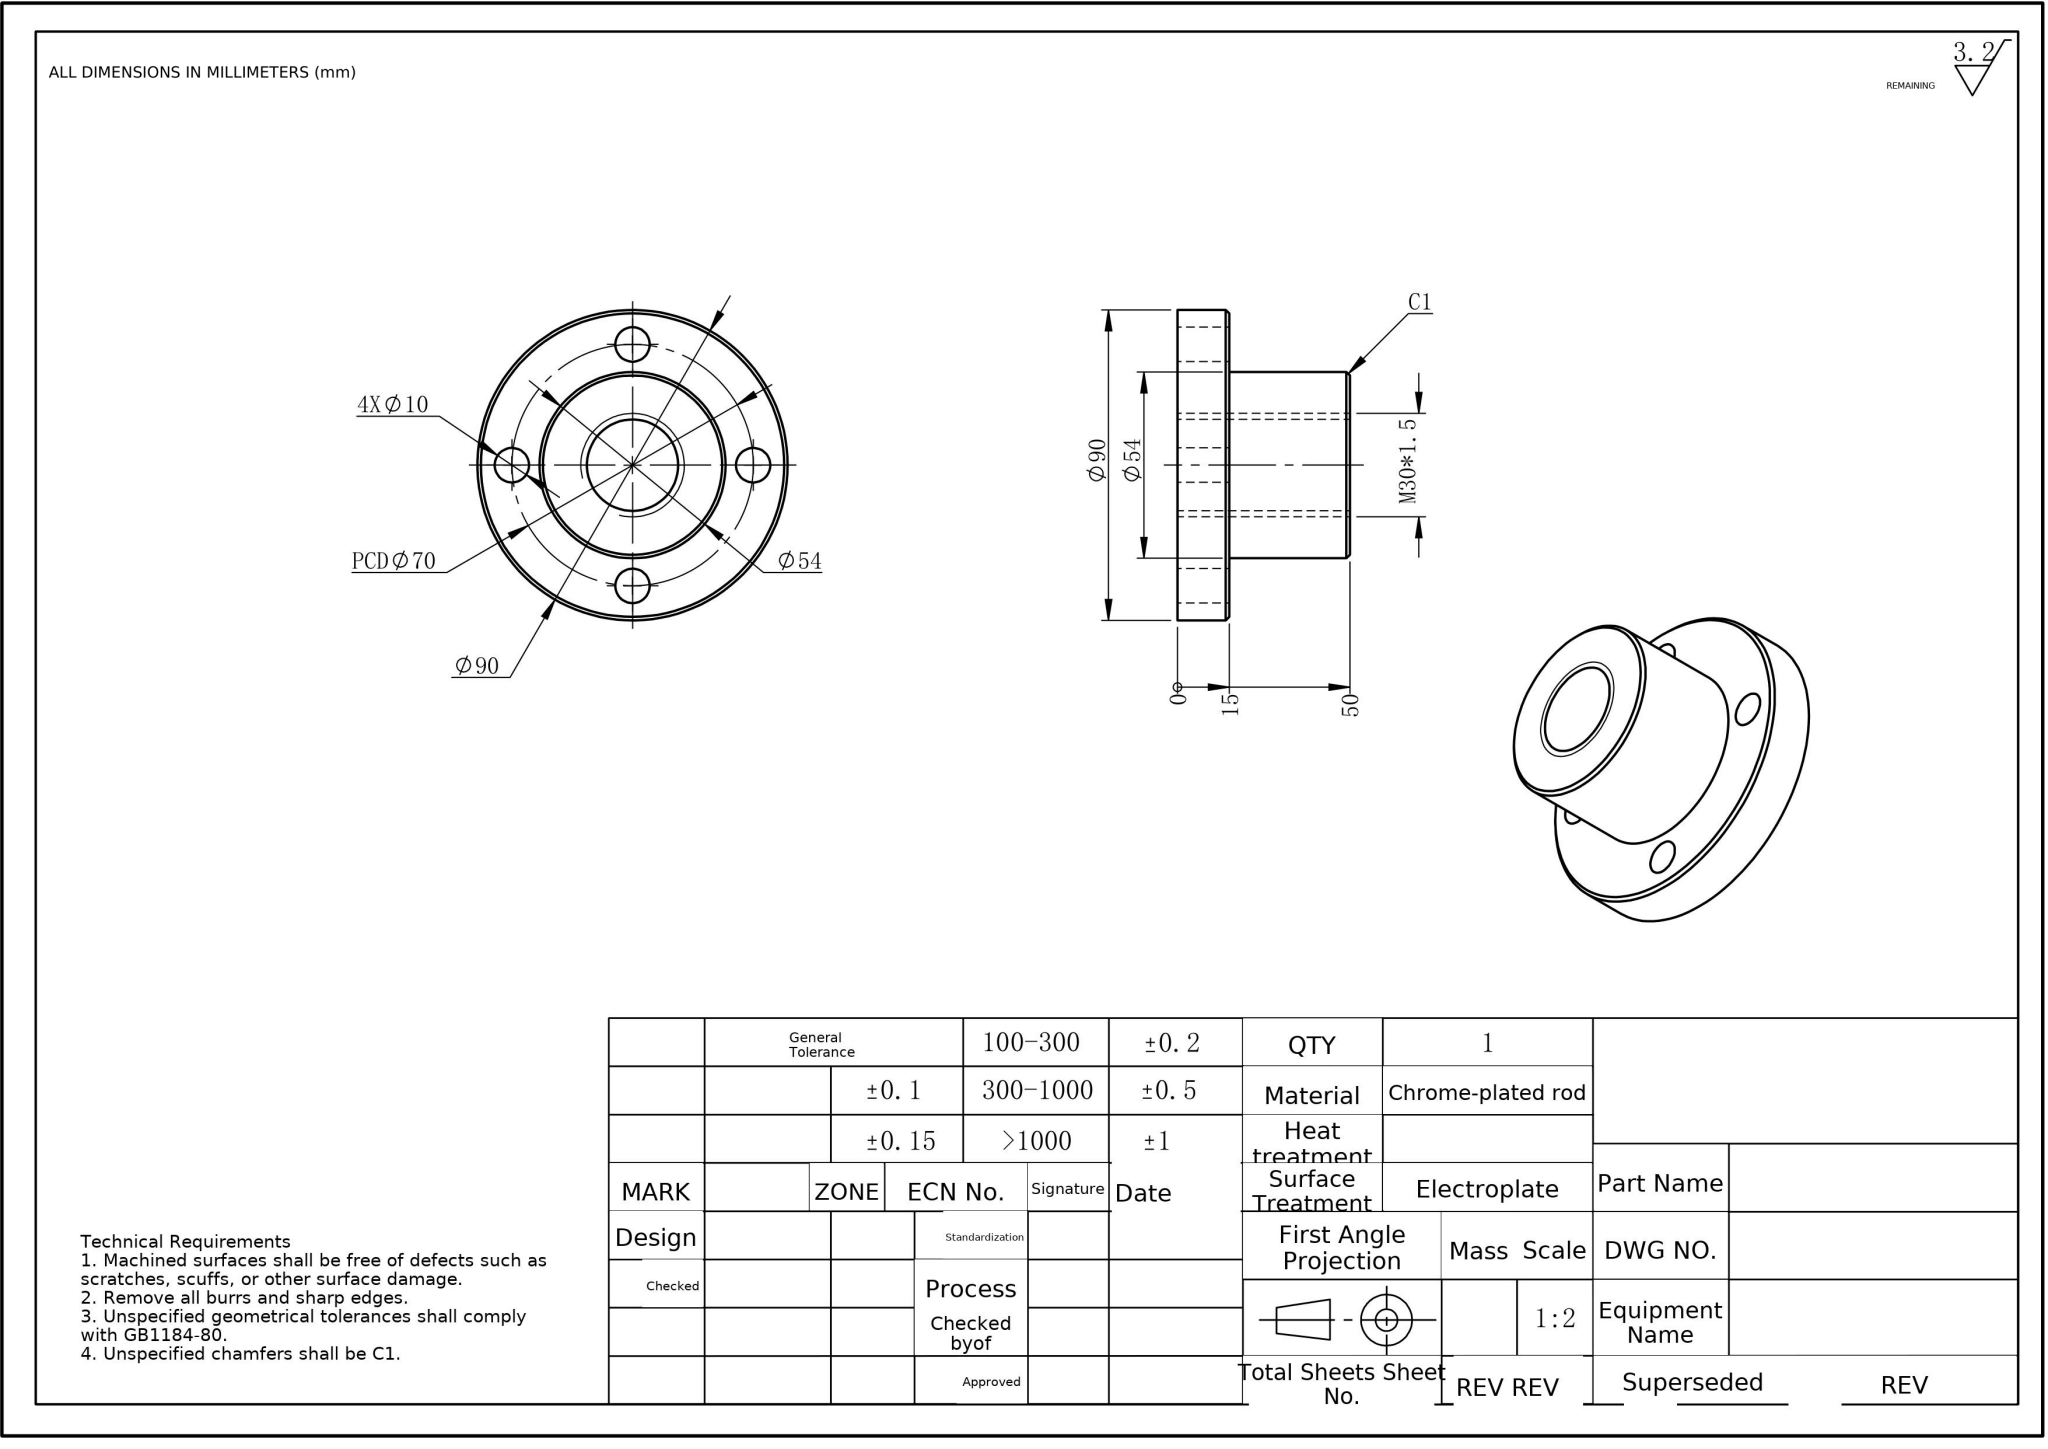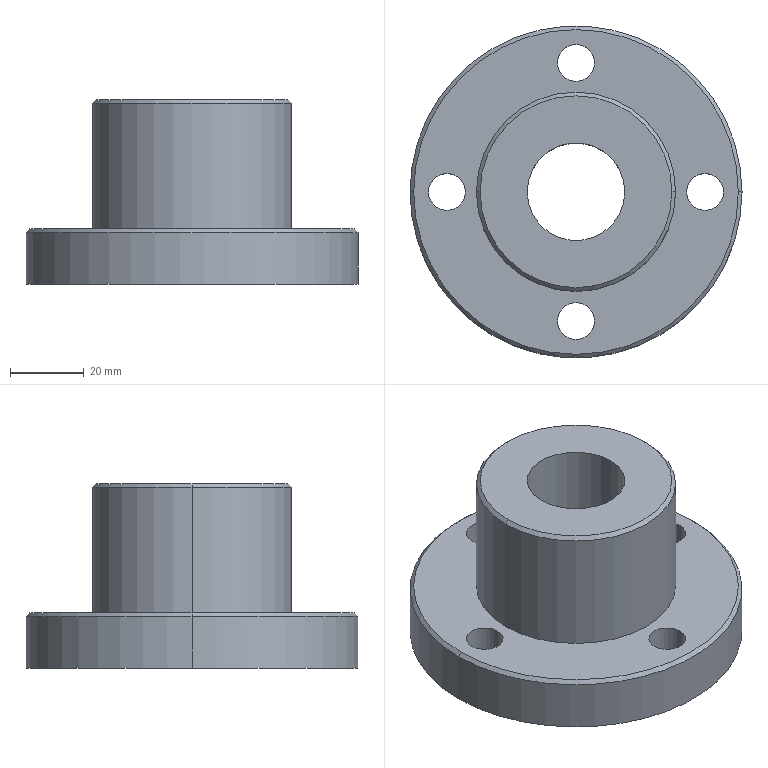Part | NX | mm | 1 solid | 21 faces | box 90 x 90 x 50 mm | volume 143070 mm3 | cylinder 14 | cone 4 | plane 3 | commonest cylinder face diameters 10 x8 26.5 x2 54 x2 90 x2
STEP:
#1=CARTESIAN_POINT('',(-13.25,0.,0.));
#2=VERTEX_POINT('',#1);
#3=CARTESIAN_POINT('',(13.25,0.,0.));
#4=VERTEX_POINT('',#3);
#5=CARTESIAN_POINT('',(0.,0.,0.));
#6=DIRECTION('',(0.,0.,1.));
#7=DIRECTION('',(1.,0.,0.));
#8=AXIS2_PLACEMENT_3D('',#5,#6,#7);
#9=CIRCLE('',#8,13.25);
#10=EDGE_CURVE('',#2,#4,#9,.T.);
#11=ORIENTED_EDGE('',*,*,#10,.F.);
#12=CARTESIAN_POINT('',(-13.25,0.,50.));
#13=VERTEX_POINT('',#12);
#14=CARTESIAN_POINT('',(-13.25,0.,50.));
#15=DIRECTION('',(0.,0.,1.));
#16=VECTOR('',#15,1000.);
#17=LINE('',#14,#16);
#18=EDGE_CURVE('',#2,#13,#17,.T.);
#19=ORIENTED_EDGE('',*,*,#18,.T.);
#20=CARTESIAN_POINT('',(13.25,0.,50.));
#21=VERTEX_POINT('',#20);
#22=CARTESIAN_POINT('',(0.,0.,50.));
#23=DIRECTION('',(0.,0.,1.));
#24=DIRECTION('',(1.,0.,0.));
#25=AXIS2_PLACEMENT_3D('',#22,#23,#24);
#26=CIRCLE('',#25,13.25);
#27=EDGE_CURVE('',#13,#21,#26,.T.);
#28=ORIENTED_EDGE('',*,*,#27,.T.);
#29=CARTESIAN_POINT('',(13.25,0.,50.));
#30=DIRECTION('',(0.,0.,1.));
#31=VECTOR('',#30,1000.);
#32=LINE('',#29,#31);
#33=EDGE_CURVE('',#4,#21,#32,.T.);
#34=ORIENTED_EDGE('',*,*,#33,.F.);
#35=EDGE_LOOP('',(#11,#19,#28,#34));
#36=FACE_OUTER_BOUND('',#35,.T.);
#37=CARTESIAN_POINT('',(0.,0.,50.));
#38=DIRECTION('',(0.,0.,1.));
#39=DIRECTION('',(1.,0.,0.));
#40=AXIS2_PLACEMENT_3D('',#37,#38,#39);
#41=CYLINDRICAL_SURFACE('',#40,13.25);
#42=ADVANCED_FACE('',(#36),#41,.F.);
#43=CARTESIAN_POINT('',(26.,0.,50.));
#44=VERTEX_POINT('',#43);
#45=CARTESIAN_POINT('',(-26.,0.,50.));
#46=VERTEX_POINT('',#45);
#47=CARTESIAN_POINT('',(0.,0.,50.));
#48=DIRECTION('',(0.,0.,1.));
#49=DIRECTION('',(1.,0.,0.));
#50=AXIS2_PLACEMENT_3D('',#47,#48,#49);
#51=CIRCLE('',#50,26.);
#52=EDGE_CURVE('',#44,#46,#51,.T.);
#53=ORIENTED_EDGE('',*,*,#52,.F.);
#54=CARTESIAN_POINT('',(27.,0.,49.));
#55=VERTEX_POINT('',#54);
#56=CARTESIAN_POINT('',(26.,0.,50.));
#57=DIRECTION('',(0.7071,0.,-0.7071));
#58=VECTOR('',#57,1000.);
#59=LINE('',#56,#58);
#60=EDGE_CURVE('',#44,#55,#59,.T.);
#61=ORIENTED_EDGE('',*,*,#60,.T.);
#62=CARTESIAN_POINT('',(-27.,0.,49.));
#63=VERTEX_POINT('',#62);
#64=CARTESIAN_POINT('',(0.,0.,49.));
#65=DIRECTION('',(0.,0.,-1.));
#66=DIRECTION('',(1.,0.,0.));
#67=AXIS2_PLACEMENT_3D('',#64,#65,#66);
#68=CIRCLE('',#67,27.);
#69=EDGE_CURVE('',#63,#55,#68,.T.);
#70=ORIENTED_EDGE('',*,*,#69,.F.);
#71=CARTESIAN_POINT('',(-26.,0.,50.));
#72=DIRECTION('',(-0.7071,0.,-0.7071));
#73=VECTOR('',#72,1000.);
#74=LINE('',#71,#73);
#75=EDGE_CURVE('',#46,#63,#74,.T.);
#76=ORIENTED_EDGE('',*,*,#75,.F.);
#77=EDGE_LOOP('',(#53,#61,#70,#76));
#78=FACE_OUTER_BOUND('',#77,.T.);
#79=CARTESIAN_POINT('',(0.,0.,50.));
#80=DIRECTION('',(0.,0.,-1.));
#81=DIRECTION('',(-1.,0.,0.));
#82=AXIS2_PLACEMENT_3D('',#79,#80,#81);
#83=CONICAL_SURFACE('',#82,26.,0.7854);
#84=ADVANCED_FACE('',(#78),#83,.T.);
#85=CARTESIAN_POINT('',(44.,0.,15.));
#86=VERTEX_POINT('',#85);
#87=CARTESIAN_POINT('',(-44.,0.,15.));
#88=VERTEX_POINT('',#87);
#89=CARTESIAN_POINT('',(0.,0.,15.));
#90=DIRECTION('',(0.,0.,1.));
#91=DIRECTION('',(1.,0.,0.));
#92=AXIS2_PLACEMENT_3D('',#89,#90,#91);
#93=CIRCLE('',#92,44.);
#94=EDGE_CURVE('',#86,#88,#93,.T.);
#95=ORIENTED_EDGE('',*,*,#94,.F.);
#96=CARTESIAN_POINT('',(45.,0.,14.));
#97=VERTEX_POINT('',#96);
#98=CARTESIAN_POINT('',(44.,0.,15.));
#99=DIRECTION('',(0.7071,0.,-0.7071));
#100=VECTOR('',#99,1000.);
#101=LINE('',#98,#100);
#102=EDGE_CURVE('',#86,#97,#101,.T.);
#103=ORIENTED_EDGE('',*,*,#102,.T.);
#104=CARTESIAN_POINT('',(-45.,0.,14.));
#105=VERTEX_POINT('',#104);
#106=CARTESIAN_POINT('',(0.,0.,14.));
#107=DIRECTION('',(0.,0.,-1.));
#108=DIRECTION('',(1.,0.,0.));
#109=AXIS2_PLACEMENT_3D('',#106,#107,#108);
#110=CIRCLE('',#109,45.);
#111=EDGE_CURVE('',#105,#97,#110,.T.);
#112=ORIENTED_EDGE('',*,*,#111,.F.);
#113=CARTESIAN_POINT('',(-44.,0.,15.));
#114=DIRECTION('',(-0.7071,0.,-0.7071));
#115=VECTOR('',#114,1000.);
#116=LINE('',#113,#115);
#117=EDGE_CURVE('',#88,#105,#116,.T.);
#118=ORIENTED_EDGE('',*,*,#117,.F.);
#119=EDGE_LOOP('',(#95,#103,#112,#118));
#120=FACE_OUTER_BOUND('',#119,.T.);
#121=CARTESIAN_POINT('',(0.,0.,15.));
#122=DIRECTION('',(0.,0.,-1.));
#123=DIRECTION('',(-1.,0.,0.));
#124=AXIS2_PLACEMENT_3D('',#121,#122,#123);
#125=CONICAL_SURFACE('',#124,44.,0.7854);
#126=ADVANCED_FACE('',(#120),#125,.T.);
#127=CARTESIAN_POINT('',(-5.,35.,0.));
#128=VERTEX_POINT('',#127);
#129=CARTESIAN_POINT('',(5.,35.,0.));
#130=VERTEX_POINT('',#129);
#131=CARTESIAN_POINT('',(-0.,35.,0.));
#132=DIRECTION('',(0.,0.,1.));
#133=DIRECTION('',(1.,0.,0.));
#134=AXIS2_PLACEMENT_3D('',#131,#132,#133);
#135=CIRCLE('',#134,5.);
#136=EDGE_CURVE('',#128,#130,#135,.T.);
#137=ORIENTED_EDGE('',*,*,#136,.F.);
#138=CARTESIAN_POINT('',(-5.,35.,15.));
#139=VERTEX_POINT('',#138);
#140=CARTESIAN_POINT('',(-5.,35.,0.));
#141=DIRECTION('',(0.,0.,1.));
#142=VECTOR('',#141,1000.);
#143=LINE('',#140,#142);
#144=EDGE_CURVE('',#128,#139,#143,.T.);
#145=ORIENTED_EDGE('',*,*,#144,.T.);
#146=CARTESIAN_POINT('',(5.,35.,15.));
#147=VERTEX_POINT('',#146);
#148=CARTESIAN_POINT('',(-0.,35.,15.));
#149=DIRECTION('',(0.,0.,1.));
#150=DIRECTION('',(1.,0.,0.));
#151=AXIS2_PLACEMENT_3D('',#148,#149,#150);
#152=CIRCLE('',#151,5.);
#153=EDGE_CURVE('',#139,#147,#152,.T.);
#154=ORIENTED_EDGE('',*,*,#153,.T.);
#155=CARTESIAN_POINT('',(5.,35.,0.));
#156=DIRECTION('',(0.,0.,1.));
#157=VECTOR('',#156,1000.);
#158=LINE('',#155,#157);
#159=EDGE_CURVE('',#130,#147,#158,.T.);
#160=ORIENTED_EDGE('',*,*,#159,.F.);
#161=EDGE_LOOP('',(#137,#145,#154,#160));
#162=FACE_OUTER_BOUND('',#161,.T.);
#163=CARTESIAN_POINT('',(-0.,35.,0.));
#164=DIRECTION('',(0.,0.,1.));
#165=DIRECTION('',(1.,0.,0.));
#166=AXIS2_PLACEMENT_3D('',#163,#164,#165);
#167=CYLINDRICAL_SURFACE('',#166,5.);
#168=ADVANCED_FACE('',(#162),#167,.F.);
#169=CARTESIAN_POINT('',(-5.,-35.,0.));
#170=VERTEX_POINT('',#169);
#171=CARTESIAN_POINT('',(5.,-35.,0.));
#172=VERTEX_POINT('',#171);
#173=CARTESIAN_POINT('',(0.,-35.,0.));
#174=DIRECTION('',(0.,0.,1.));
#175=DIRECTION('',(1.,0.,0.));
#176=AXIS2_PLACEMENT_3D('',#173,#174,#175);
#177=CIRCLE('',#176,5.);
#178=EDGE_CURVE('',#170,#172,#177,.T.);
#179=ORIENTED_EDGE('',*,*,#178,.F.);
#180=CARTESIAN_POINT('',(-5.,-35.,15.));
#181=VERTEX_POINT('',#180);
#182=CARTESIAN_POINT('',(-5.,-35.,0.));
#183=DIRECTION('',(0.,0.,1.));
#184=VECTOR('',#183,1000.);
#185=LINE('',#182,#184);
#186=EDGE_CURVE('',#170,#181,#185,.T.);
#187=ORIENTED_EDGE('',*,*,#186,.T.);
#188=CARTESIAN_POINT('',(5.,-35.,15.));
#189=VERTEX_POINT('',#188);
#190=CARTESIAN_POINT('',(0.,-35.,15.));
#191=DIRECTION('',(0.,0.,1.));
#192=DIRECTION('',(1.,0.,0.));
#193=AXIS2_PLACEMENT_3D('',#190,#191,#192);
#194=CIRCLE('',#193,5.);
#195=EDGE_CURVE('',#181,#189,#194,.T.);
#196=ORIENTED_EDGE('',*,*,#195,.T.);
#197=CARTESIAN_POINT('',(5.,-35.,0.));
#198=DIRECTION('',(0.,0.,1.));
#199=VECTOR('',#198,1000.);
#200=LINE('',#197,#199);
#201=EDGE_CURVE('',#172,#189,#200,.T.);
#202=ORIENTED_EDGE('',*,*,#201,.F.);
#203=EDGE_LOOP('',(#179,#187,#196,#202));
#204=FACE_OUTER_BOUND('',#203,.T.);
#205=CARTESIAN_POINT('',(0.,-35.,0.));
#206=DIRECTION('',(0.,0.,1.));
#207=DIRECTION('',(1.,0.,0.));
#208=AXIS2_PLACEMENT_3D('',#205,#206,#207);
#209=CYLINDRICAL_SURFACE('',#208,5.);
#210=ADVANCED_FACE('',(#204),#209,.F.);
#211=CARTESIAN_POINT('',(-40.,-0.,0.));
#212=VERTEX_POINT('',#211);
#213=CARTESIAN_POINT('',(-30.,-0.,0.));
#214=VERTEX_POINT('',#213);
#215=CARTESIAN_POINT('',(-35.,-0.,0.));
#216=DIRECTION('',(0.,0.,1.));
#217=DIRECTION('',(1.,0.,0.));
#218=AXIS2_PLACEMENT_3D('',#215,#216,#217);
#219=CIRCLE('',#218,5.);
#220=EDGE_CURVE('',#212,#214,#219,.T.);
#221=ORIENTED_EDGE('',*,*,#220,.F.);
#222=CARTESIAN_POINT('',(-40.,-0.,15.));
#223=VERTEX_POINT('',#222);
#224=CARTESIAN_POINT('',(-40.,-0.,0.));
#225=DIRECTION('',(0.,0.,1.));
#226=VECTOR('',#225,1000.);
#227=LINE('',#224,#226);
#228=EDGE_CURVE('',#212,#223,#227,.T.);
#229=ORIENTED_EDGE('',*,*,#228,.T.);
#230=CARTESIAN_POINT('',(-30.,-0.,15.));
#231=VERTEX_POINT('',#230);
#232=CARTESIAN_POINT('',(-35.,-0.,15.));
#233=DIRECTION('',(0.,0.,1.));
#234=DIRECTION('',(1.,0.,0.));
#235=AXIS2_PLACEMENT_3D('',#232,#233,#234);
#236=CIRCLE('',#235,5.);
#237=EDGE_CURVE('',#223,#231,#236,.T.);
#238=ORIENTED_EDGE('',*,*,#237,.T.);
#239=CARTESIAN_POINT('',(-30.,-0.,0.));
#240=DIRECTION('',(0.,0.,1.));
#241=VECTOR('',#240,1000.);
#242=LINE('',#239,#241);
#243=EDGE_CURVE('',#214,#231,#242,.T.);
#244=ORIENTED_EDGE('',*,*,#243,.F.);
#245=EDGE_LOOP('',(#221,#229,#238,#244));
#246=FACE_OUTER_BOUND('',#245,.T.);
#247=CARTESIAN_POINT('',(-35.,-0.,0.));
#248=DIRECTION('',(0.,0.,1.));
#249=DIRECTION('',(1.,0.,0.));
#250=AXIS2_PLACEMENT_3D('',#247,#248,#249);
#251=CYLINDRICAL_SURFACE('',#250,5.);
#252=ADVANCED_FACE('',(#246),#251,.F.);
#253=CARTESIAN_POINT('',(30.,0.,0.));
#254=VERTEX_POINT('',#253);
#255=CARTESIAN_POINT('',(40.,0.,0.));
#256=VERTEX_POINT('',#255);
#257=CARTESIAN_POINT('',(35.,0.,0.));
#258=DIRECTION('',(0.,0.,1.));
#259=DIRECTION('',(1.,0.,0.));
#260=AXIS2_PLACEMENT_3D('',#257,#258,#259);
#261=CIRCLE('',#260,5.);
#262=EDGE_CURVE('',#254,#256,#261,.T.);
#263=ORIENTED_EDGE('',*,*,#262,.F.);
#264=CARTESIAN_POINT('',(30.,0.,15.));
#265=VERTEX_POINT('',#264);
#266=CARTESIAN_POINT('',(30.,0.,0.));
#267=DIRECTION('',(0.,0.,1.));
#268=VECTOR('',#267,1000.);
#269=LINE('',#266,#268);
#270=EDGE_CURVE('',#254,#265,#269,.T.);
#271=ORIENTED_EDGE('',*,*,#270,.T.);
#272=CARTESIAN_POINT('',(40.,0.,15.));
#273=VERTEX_POINT('',#272);
#274=CARTESIAN_POINT('',(35.,0.,15.));
#275=DIRECTION('',(0.,0.,1.));
#276=DIRECTION('',(1.,0.,0.));
#277=AXIS2_PLACEMENT_3D('',#274,#275,#276);
#278=CIRCLE('',#277,5.);
#279=EDGE_CURVE('',#265,#273,#278,.T.);
#280=ORIENTED_EDGE('',*,*,#279,.T.);
#281=CARTESIAN_POINT('',(40.,0.,0.));
#282=DIRECTION('',(0.,0.,1.));
#283=VECTOR('',#282,1000.);
#284=LINE('',#281,#283);
#285=EDGE_CURVE('',#256,#273,#284,.T.);
#286=ORIENTED_EDGE('',*,*,#285,.F.);
#287=EDGE_LOOP('',(#263,#271,#280,#286));
#288=FACE_OUTER_BOUND('',#287,.T.);
#289=CARTESIAN_POINT('',(35.,0.,0.));
#290=DIRECTION('',(0.,0.,1.));
#291=DIRECTION('',(1.,0.,0.));
#292=AXIS2_PLACEMENT_3D('',#289,#290,#291);
#293=CYLINDRICAL_SURFACE('',#292,5.);
#294=ADVANCED_FACE('',(#288),#293,.F.);
#295=ORIENTED_EDGE('',*,*,#69,.T.);
#296=CARTESIAN_POINT('',(27.,0.,15.));
#297=VERTEX_POINT('',#296);
#298=CARTESIAN_POINT('',(27.,0.,50.));
#299=DIRECTION('',(0.,0.,-1.));
#300=VECTOR('',#299,1000.);
#301=LINE('',#298,#300);
#302=EDGE_CURVE('',#55,#297,#301,.T.);
#303=ORIENTED_EDGE('',*,*,#302,.T.);
#304=CARTESIAN_POINT('',(-27.,0.,15.));
#305=VERTEX_POINT('',#304);
#306=CARTESIAN_POINT('',(0.,0.,15.));
#307=DIRECTION('',(0.,0.,1.));
#308=DIRECTION('',(1.,0.,0.));
#309=AXIS2_PLACEMENT_3D('',#306,#307,#308);
#310=CIRCLE('',#309,27.);
#311=EDGE_CURVE('',#297,#305,#310,.T.);
#312=ORIENTED_EDGE('',*,*,#311,.T.);
#313=CARTESIAN_POINT('',(-27.,0.,50.));
#314=DIRECTION('',(0.,0.,-1.));
#315=VECTOR('',#314,1000.);
#316=LINE('',#313,#315);
#317=EDGE_CURVE('',#63,#305,#316,.T.);
#318=ORIENTED_EDGE('',*,*,#317,.F.);
#319=EDGE_LOOP('',(#295,#303,#312,#318));
#320=FACE_OUTER_BOUND('',#319,.T.);
#321=CARTESIAN_POINT('',(0.,0.,50.));
#322=DIRECTION('',(0.,0.,-1.));
#323=DIRECTION('',(-1.,0.,0.));
#324=AXIS2_PLACEMENT_3D('',#321,#322,#323);
#325=CYLINDRICAL_SURFACE('',#324,27.);
#326=ADVANCED_FACE('',(#320),#325,.T.);
#327=ORIENTED_EDGE('',*,*,#111,.T.);
#328=CARTESIAN_POINT('',(45.,0.,0.));
#329=VERTEX_POINT('',#328);
#330=CARTESIAN_POINT('',(45.,0.,15.));
#331=DIRECTION('',(0.,0.,-1.));
#332=VECTOR('',#331,1000.);
#333=LINE('',#330,#332);
#334=EDGE_CURVE('',#97,#329,#333,.T.);
#335=ORIENTED_EDGE('',*,*,#334,.T.);
#336=CARTESIAN_POINT('',(-45.,0.,0.));
#337=VERTEX_POINT('',#336);
#338=CARTESIAN_POINT('',(0.,0.,0.));
#339=DIRECTION('',(0.,0.,1.));
#340=DIRECTION('',(1.,0.,0.));
#341=AXIS2_PLACEMENT_3D('',#338,#339,#340);
#342=CIRCLE('',#341,45.);
#343=EDGE_CURVE('',#329,#337,#342,.T.);
#344=ORIENTED_EDGE('',*,*,#343,.T.);
#345=CARTESIAN_POINT('',(-45.,0.,15.));
#346=DIRECTION('',(0.,0.,-1.));
#347=VECTOR('',#346,1000.);
#348=LINE('',#345,#347);
#349=EDGE_CURVE('',#105,#337,#348,.T.);
#350=ORIENTED_EDGE('',*,*,#349,.F.);
#351=EDGE_LOOP('',(#327,#335,#344,#350));
#352=FACE_OUTER_BOUND('',#351,.T.);
#353=CARTESIAN_POINT('',(0.,0.,15.));
#354=DIRECTION('',(0.,0.,-1.));
#355=DIRECTION('',(-1.,0.,0.));
#356=AXIS2_PLACEMENT_3D('',#353,#354,#355);
#357=CYLINDRICAL_SURFACE('',#356,45.);
#358=ADVANCED_FACE('',(#352),#357,.T.);
#359=ORIENTED_EDGE('',*,*,#334,.F.);
#360=CARTESIAN_POINT('',(0.,0.,14.));
#361=DIRECTION('',(0.,0.,-1.));
#362=DIRECTION('',(1.,0.,0.));
#363=AXIS2_PLACEMENT_3D('',#360,#361,#362);
#364=CIRCLE('',#363,45.);
#365=EDGE_CURVE('',#97,#105,#364,.T.);
#366=ORIENTED_EDGE('',*,*,#365,.T.);
#367=ORIENTED_EDGE('',*,*,#349,.T.);
#368=CARTESIAN_POINT('',(0.,0.,0.));
#369=DIRECTION('',(0.,0.,1.));
#370=DIRECTION('',(1.,0.,0.));
#371=AXIS2_PLACEMENT_3D('',#368,#369,#370);
#372=CIRCLE('',#371,45.);
#373=EDGE_CURVE('',#337,#329,#372,.T.);
#374=ORIENTED_EDGE('',*,*,#373,.T.);
#375=EDGE_LOOP('',(#359,#366,#367,#374));
#376=FACE_OUTER_BOUND('',#375,.T.);
#377=CARTESIAN_POINT('',(0.,0.,15.));
#378=DIRECTION('',(0.,0.,-1.));
#379=DIRECTION('',(-1.,0.,0.));
#380=AXIS2_PLACEMENT_3D('',#377,#378,#379);
#381=CYLINDRICAL_SURFACE('',#380,45.);
#382=ADVANCED_FACE('',(#376),#381,.T.);
#383=CARTESIAN_POINT('',(0.,0.,15.));
#384=DIRECTION('',(0.,0.,1.));
#385=DIRECTION('',(1.,0.,0.));
#386=AXIS2_PLACEMENT_3D('',#383,#384,#385);
#387=CIRCLE('',#386,44.);
#388=EDGE_CURVE('',#88,#86,#387,.T.);
#389=ORIENTED_EDGE('',*,*,#388,.T.);
#390=ORIENTED_EDGE('',*,*,#94,.T.);
#391=EDGE_LOOP('',(#389,#390));
#392=FACE_OUTER_BOUND('',#391,.T.);
#393=CARTESIAN_POINT('',(-0.,35.,15.));
#394=DIRECTION('',(0.,0.,1.));
#395=DIRECTION('',(1.,0.,0.));
#396=AXIS2_PLACEMENT_3D('',#393,#394,#395);
#397=CIRCLE('',#396,5.);
#398=EDGE_CURVE('',#147,#139,#397,.T.);
#399=ORIENTED_EDGE('',*,*,#398,.F.);
#400=ORIENTED_EDGE('',*,*,#153,.F.);
#401=EDGE_LOOP('',(#399,#400));
#402=FACE_BOUND('',#401,.T.);
#403=CARTESIAN_POINT('',(0.,-35.,15.));
#404=DIRECTION('',(0.,0.,1.));
#405=DIRECTION('',(1.,0.,0.));
#406=AXIS2_PLACEMENT_3D('',#403,#404,#405);
#407=CIRCLE('',#406,5.);
#408=EDGE_CURVE('',#189,#181,#407,.T.);
#409=ORIENTED_EDGE('',*,*,#408,.F.);
#410=ORIENTED_EDGE('',*,*,#195,.F.);
#411=EDGE_LOOP('',(#409,#410));
#412=FACE_BOUND('',#411,.T.);
#413=CARTESIAN_POINT('',(-35.,-0.,15.));
#414=DIRECTION('',(0.,0.,1.));
#415=DIRECTION('',(1.,0.,0.));
#416=AXIS2_PLACEMENT_3D('',#413,#414,#415);
#417=CIRCLE('',#416,5.);
#418=EDGE_CURVE('',#231,#223,#417,.T.);
#419=ORIENTED_EDGE('',*,*,#418,.F.);
#420=ORIENTED_EDGE('',*,*,#237,.F.);
#421=EDGE_LOOP('',(#419,#420));
#422=FACE_BOUND('',#421,.T.);
#423=CARTESIAN_POINT('',(35.,0.,15.));
#424=DIRECTION('',(0.,0.,1.));
#425=DIRECTION('',(1.,0.,0.));
#426=AXIS2_PLACEMENT_3D('',#423,#424,#425);
#427=CIRCLE('',#426,5.);
#428=EDGE_CURVE('',#273,#265,#427,.T.);
#429=ORIENTED_EDGE('',*,*,#428,.F.);
#430=ORIENTED_EDGE('',*,*,#279,.F.);
#431=EDGE_LOOP('',(#429,#430));
#432=FACE_BOUND('',#431,.T.);
#433=CARTESIAN_POINT('',(0.,0.,15.));
#434=DIRECTION('',(0.,0.,1.));
#435=DIRECTION('',(1.,0.,0.));
#436=AXIS2_PLACEMENT_3D('',#433,#434,#435);
#437=CIRCLE('',#436,27.);
#438=EDGE_CURVE('',#305,#297,#437,.T.);
#439=ORIENTED_EDGE('',*,*,#438,.F.);
#440=ORIENTED_EDGE('',*,*,#311,.F.);
#441=EDGE_LOOP('',(#439,#440));
#442=FACE_BOUND('',#441,.T.);
#443=CARTESIAN_POINT('',(0.,0.,15.));
#444=DIRECTION('',(0.,0.,1.));
#445=DIRECTION('',(1.,0.,0.));
#446=AXIS2_PLACEMENT_3D('',#443,#444,#445);
#447=PLANE('',#446);
#448=ADVANCED_FACE('',(#392,#402,#412,#422,#432,#442),#447,.T.);
#449=CARTESIAN_POINT('',(0.,0.,0.));
#450=DIRECTION('',(0.,0.,1.));
#451=DIRECTION('',(1.,0.,0.));
#452=AXIS2_PLACEMENT_3D('',#449,#450,#451);
#453=CIRCLE('',#452,13.25);
#454=EDGE_CURVE('',#4,#2,#453,.T.);
#455=ORIENTED_EDGE('',*,*,#454,.T.);
#456=ORIENTED_EDGE('',*,*,#10,.T.);
#457=EDGE_LOOP('',(#455,#456));
#458=FACE_BOUND('',#457,.T.);
#459=CARTESIAN_POINT('',(-0.,35.,0.));
#460=DIRECTION('',(0.,0.,1.));
#461=DIRECTION('',(1.,0.,0.));
#462=AXIS2_PLACEMENT_3D('',#459,#460,#461);
#463=CIRCLE('',#462,5.);
#464=EDGE_CURVE('',#130,#128,#463,.T.);
#465=ORIENTED_EDGE('',*,*,#464,.T.);
#466=ORIENTED_EDGE('',*,*,#136,.T.);
#467=EDGE_LOOP('',(#465,#466));
#468=FACE_BOUND('',#467,.T.);
#469=CARTESIAN_POINT('',(0.,-35.,0.));
#470=DIRECTION('',(0.,0.,1.));
#471=DIRECTION('',(1.,0.,0.));
#472=AXIS2_PLACEMENT_3D('',#469,#470,#471);
#473=CIRCLE('',#472,5.);
#474=EDGE_CURVE('',#172,#170,#473,.T.);
#475=ORIENTED_EDGE('',*,*,#474,.T.);
#476=ORIENTED_EDGE('',*,*,#178,.T.);
#477=EDGE_LOOP('',(#475,#476));
#478=FACE_BOUND('',#477,.T.);
#479=CARTESIAN_POINT('',(-35.,-0.,0.));
#480=DIRECTION('',(0.,0.,1.));
#481=DIRECTION('',(1.,0.,0.));
#482=AXIS2_PLACEMENT_3D('',#479,#480,#481);
#483=CIRCLE('',#482,5.);
#484=EDGE_CURVE('',#214,#212,#483,.T.);
#485=ORIENTED_EDGE('',*,*,#484,.T.);
#486=ORIENTED_EDGE('',*,*,#220,.T.);
#487=EDGE_LOOP('',(#485,#486));
#488=FACE_BOUND('',#487,.T.);
#489=CARTESIAN_POINT('',(35.,0.,0.));
#490=DIRECTION('',(0.,0.,1.));
#491=DIRECTION('',(1.,0.,0.));
#492=AXIS2_PLACEMENT_3D('',#489,#490,#491);
#493=CIRCLE('',#492,5.);
#494=EDGE_CURVE('',#256,#254,#493,.T.);
#495=ORIENTED_EDGE('',*,*,#494,.T.);
#496=ORIENTED_EDGE('',*,*,#262,.T.);
#497=EDGE_LOOP('',(#495,#496));
#498=FACE_BOUND('',#497,.T.);
#499=ORIENTED_EDGE('',*,*,#373,.F.);
#500=ORIENTED_EDGE('',*,*,#343,.F.);
#501=EDGE_LOOP('',(#499,#500));
#502=FACE_OUTER_BOUND('',#501,.T.);
#503=CARTESIAN_POINT('',(0.,0.,0.));
#504=DIRECTION('',(0.,0.,1.));
#505=DIRECTION('',(1.,0.,0.));
#506=AXIS2_PLACEMENT_3D('',#503,#504,#505);
#507=PLANE('',#506);
#508=ADVANCED_FACE('',(#458,#468,#478,#488,#498,#502),#507,.F.);
#509=CARTESIAN_POINT('',(0.,0.,50.));
#510=DIRECTION('',(0.,0.,1.));
#511=DIRECTION('',(1.,0.,0.));
#512=AXIS2_PLACEMENT_3D('',#509,#510,#511);
#513=CIRCLE('',#512,13.25);
#514=EDGE_CURVE('',#21,#13,#513,.T.);
#515=ORIENTED_EDGE('',*,*,#514,.F.);
#516=ORIENTED_EDGE('',*,*,#27,.F.);
#517=EDGE_LOOP('',(#515,#516));
#518=FACE_BOUND('',#517,.T.);
#519=CARTESIAN_POINT('',(0.,0.,50.));
#520=DIRECTION('',(0.,0.,1.));
#521=DIRECTION('',(1.,0.,0.));
#522=AXIS2_PLACEMENT_3D('',#519,#520,#521);
#523=CIRCLE('',#522,26.);
#524=EDGE_CURVE('',#46,#44,#523,.T.);
#525=ORIENTED_EDGE('',*,*,#524,.T.);
#526=ORIENTED_EDGE('',*,*,#52,.T.);
#527=EDGE_LOOP('',(#525,#526));
#528=FACE_OUTER_BOUND('',#527,.T.);
#529=CARTESIAN_POINT('',(0.,0.,50.));
#530=DIRECTION('',(0.,0.,1.));
#531=DIRECTION('',(1.,0.,0.));
#532=AXIS2_PLACEMENT_3D('',#529,#530,#531);
#533=PLANE('',#532);
#534=ADVANCED_FACE('',(#518,#528),#533,.T.);
#535=ORIENTED_EDGE('',*,*,#302,.F.);
#536=CARTESIAN_POINT('',(0.,0.,49.));
#537=DIRECTION('',(0.,0.,-1.));
#538=DIRECTION('',(1.,0.,0.));
#539=AXIS2_PLACEMENT_3D('',#536,#537,#538);
#540=CIRCLE('',#539,27.);
#541=EDGE_CURVE('',#55,#63,#540,.T.);
#542=ORIENTED_EDGE('',*,*,#541,.T.);
#543=ORIENTED_EDGE('',*,*,#317,.T.);
#544=ORIENTED_EDGE('',*,*,#438,.T.);
#545=EDGE_LOOP('',(#535,#542,#543,#544));
#546=FACE_OUTER_BOUND('',#545,.T.);
#547=CARTESIAN_POINT('',(0.,0.,50.));
#548=DIRECTION('',(0.,0.,-1.));
#549=DIRECTION('',(-1.,0.,0.));
#550=AXIS2_PLACEMENT_3D('',#547,#548,#549);
#551=CYLINDRICAL_SURFACE('',#550,27.);
#552=ADVANCED_FACE('',(#546),#551,.T.);
#553=ORIENTED_EDGE('',*,*,#270,.F.);
#554=ORIENTED_EDGE('',*,*,#494,.F.);
#555=ORIENTED_EDGE('',*,*,#285,.T.);
#556=ORIENTED_EDGE('',*,*,#428,.T.);
#557=EDGE_LOOP('',(#553,#554,#555,#556));
#558=FACE_OUTER_BOUND('',#557,.T.);
#559=CARTESIAN_POINT('',(35.,0.,0.));
#560=DIRECTION('',(0.,0.,1.));
#561=DIRECTION('',(1.,0.,0.));
#562=AXIS2_PLACEMENT_3D('',#559,#560,#561);
#563=CYLINDRICAL_SURFACE('',#562,5.);
#564=ADVANCED_FACE('',(#558),#563,.F.);
#565=ORIENTED_EDGE('',*,*,#228,.F.);
#566=ORIENTED_EDGE('',*,*,#484,.F.);
#567=ORIENTED_EDGE('',*,*,#243,.T.);
#568=ORIENTED_EDGE('',*,*,#418,.T.);
#569=EDGE_LOOP('',(#565,#566,#567,#568));
#570=FACE_OUTER_BOUND('',#569,.T.);
#571=CARTESIAN_POINT('',(-35.,-0.,0.));
#572=DIRECTION('',(0.,0.,1.));
#573=DIRECTION('',(1.,0.,0.));
#574=AXIS2_PLACEMENT_3D('',#571,#572,#573);
#575=CYLINDRICAL_SURFACE('',#574,5.);
#576=ADVANCED_FACE('',(#570),#575,.F.);
#577=ORIENTED_EDGE('',*,*,#186,.F.);
#578=ORIENTED_EDGE('',*,*,#474,.F.);
#579=ORIENTED_EDGE('',*,*,#201,.T.);
#580=ORIENTED_EDGE('',*,*,#408,.T.);
#581=EDGE_LOOP('',(#577,#578,#579,#580));
#582=FACE_OUTER_BOUND('',#581,.T.);
#583=CARTESIAN_POINT('',(0.,-35.,0.));
#584=DIRECTION('',(0.,0.,1.));
#585=DIRECTION('',(1.,0.,0.));
#586=AXIS2_PLACEMENT_3D('',#583,#584,#585);
#587=CYLINDRICAL_SURFACE('',#586,5.);
#588=ADVANCED_FACE('',(#582),#587,.F.);
#589=ORIENTED_EDGE('',*,*,#144,.F.);
#590=ORIENTED_EDGE('',*,*,#464,.F.);
#591=ORIENTED_EDGE('',*,*,#159,.T.);
#592=ORIENTED_EDGE('',*,*,#398,.T.);
#593=EDGE_LOOP('',(#589,#590,#591,#592));
#594=FACE_OUTER_BOUND('',#593,.T.);
#595=CARTESIAN_POINT('',(-0.,35.,0.));
#596=DIRECTION('',(0.,0.,1.));
#597=DIRECTION('',(1.,0.,0.));
#598=AXIS2_PLACEMENT_3D('',#595,#596,#597);
#599=CYLINDRICAL_SURFACE('',#598,5.);
#600=ADVANCED_FACE('',(#594),#599,.F.);
#601=ORIENTED_EDGE('',*,*,#102,.F.);
#602=ORIENTED_EDGE('',*,*,#388,.F.);
#603=ORIENTED_EDGE('',*,*,#117,.T.);
#604=ORIENTED_EDGE('',*,*,#365,.F.);
#605=EDGE_LOOP('',(#601,#602,#603,#604));
#606=FACE_OUTER_BOUND('',#605,.T.);
#607=CARTESIAN_POINT('',(0.,0.,15.));
#608=DIRECTION('',(0.,0.,-1.));
#609=DIRECTION('',(-1.,0.,0.));
#610=AXIS2_PLACEMENT_3D('',#607,#608,#609);
#611=CONICAL_SURFACE('',#610,44.,0.7854);
#612=ADVANCED_FACE('',(#606),#611,.T.);
#613=ORIENTED_EDGE('',*,*,#60,.F.);
#614=ORIENTED_EDGE('',*,*,#524,.F.);
#615=ORIENTED_EDGE('',*,*,#75,.T.);
#616=ORIENTED_EDGE('',*,*,#541,.F.);
#617=EDGE_LOOP('',(#613,#614,#615,#616));
#618=FACE_OUTER_BOUND('',#617,.T.);
#619=CARTESIAN_POINT('',(0.,0.,50.));
#620=DIRECTION('',(0.,0.,-1.));
#621=DIRECTION('',(-1.,0.,0.));
#622=AXIS2_PLACEMENT_3D('',#619,#620,#621);
#623=CONICAL_SURFACE('',#622,26.,0.7854);
#624=ADVANCED_FACE('',(#618),#623,.T.);
#625=ORIENTED_EDGE('',*,*,#18,.F.);
#626=ORIENTED_EDGE('',*,*,#454,.F.);
#627=ORIENTED_EDGE('',*,*,#33,.T.);
#628=ORIENTED_EDGE('',*,*,#514,.T.);
#629=EDGE_LOOP('',(#625,#626,#627,#628));
#630=FACE_OUTER_BOUND('',#629,.T.);
#631=CARTESIAN_POINT('',(0.,0.,50.));
#632=DIRECTION('',(0.,0.,1.));
#633=DIRECTION('',(1.,0.,0.));
#634=AXIS2_PLACEMENT_3D('',#631,#632,#633);
#635=CYLINDRICAL_SURFACE('',#634,13.25);
#636=ADVANCED_FACE('',(#630),#635,.F.);
#637=CLOSED_SHELL('',(#42,#84,#126,#168,#210,#252,#294,#326,#358,#382,#448,#508,#534,#552,#564,#576,#588,#600,#612,#624,#636));
#638=MANIFOLD_SOLID_BREP('',#637);
#639=CARTESIAN_POINT('',(0.,0.,0.));
#640=DIRECTION('',(0.,0.,1.));
#641=DIRECTION('',(1.,0.,0.));
#642=AXIS2_PLACEMENT_3D('',#639,#640,#641);
#643=(LENGTH_UNIT()NAMED_UNIT(*)SI_UNIT(.MILLI.,.METRE.));
#644=UNCERTAINTY_MEASURE_WITH_UNIT(LENGTH_MEASURE(0.00001),#643,'','');
#645=(NAMED_UNIT(*)PLANE_ANGLE_UNIT()SI_UNIT($,.RADIAN.));
#646=(NAMED_UNIT(*)SI_UNIT($,.STERADIAN.)SOLID_ANGLE_UNIT());
#647=(GEOMETRIC_REPRESENTATION_CONTEXT(3)GLOBAL_UNCERTAINTY_ASSIGNED_CONTEXT((#644))GLOBAL_UNIT_ASSIGNED_CONTEXT((#643,#645,#646))REPRESENTATION_CONTEXT('',''));
#648=ADVANCED_BREP_SHAPE_REPRESENTATION('',(#638,#642),#647);
#649=COLOUR_RGB('',0.7922,0.8196,0.9333);
#650=FILL_AREA_STYLE_COLOUR('',#649);
#651=FILL_AREA_STYLE('',(#650));
#652=SURFACE_STYLE_FILL_AREA(#651);
#653=SURFACE_SIDE_STYLE('',(#652));
#654=SURFACE_STYLE_USAGE(.BOTH.,#653);
#655=PRESENTATION_STYLE_ASSIGNMENT((#654));
#656=STYLED_ITEM('',(#655),#638);
#657=PRESENTATION_LAYER_ASSIGNMENT('','',(#656));
#658=(LENGTH_UNIT()NAMED_UNIT(*)SI_UNIT(.MILLI.,.METRE.));
#659=UNCERTAINTY_MEASURE_WITH_UNIT(LENGTH_MEASURE(0.00001),#658,'','');
#660=(NAMED_UNIT(*)PLANE_ANGLE_UNIT()SI_UNIT($,.RADIAN.));
#661=(NAMED_UNIT(*)SI_UNIT($,.STERADIAN.)SOLID_ANGLE_UNIT());
#662=(GEOMETRIC_REPRESENTATION_CONTEXT(3)GLOBAL_UNCERTAINTY_ASSIGNED_CONTEXT((#659))GLOBAL_UNIT_ASSIGNED_CONTEXT((#658,#660,#661))REPRESENTATION_CONTEXT('',''));
#663=MECHANICAL_DESIGN_GEOMETRIC_PRESENTATION_REPRESENTATION('',(#656),#662);